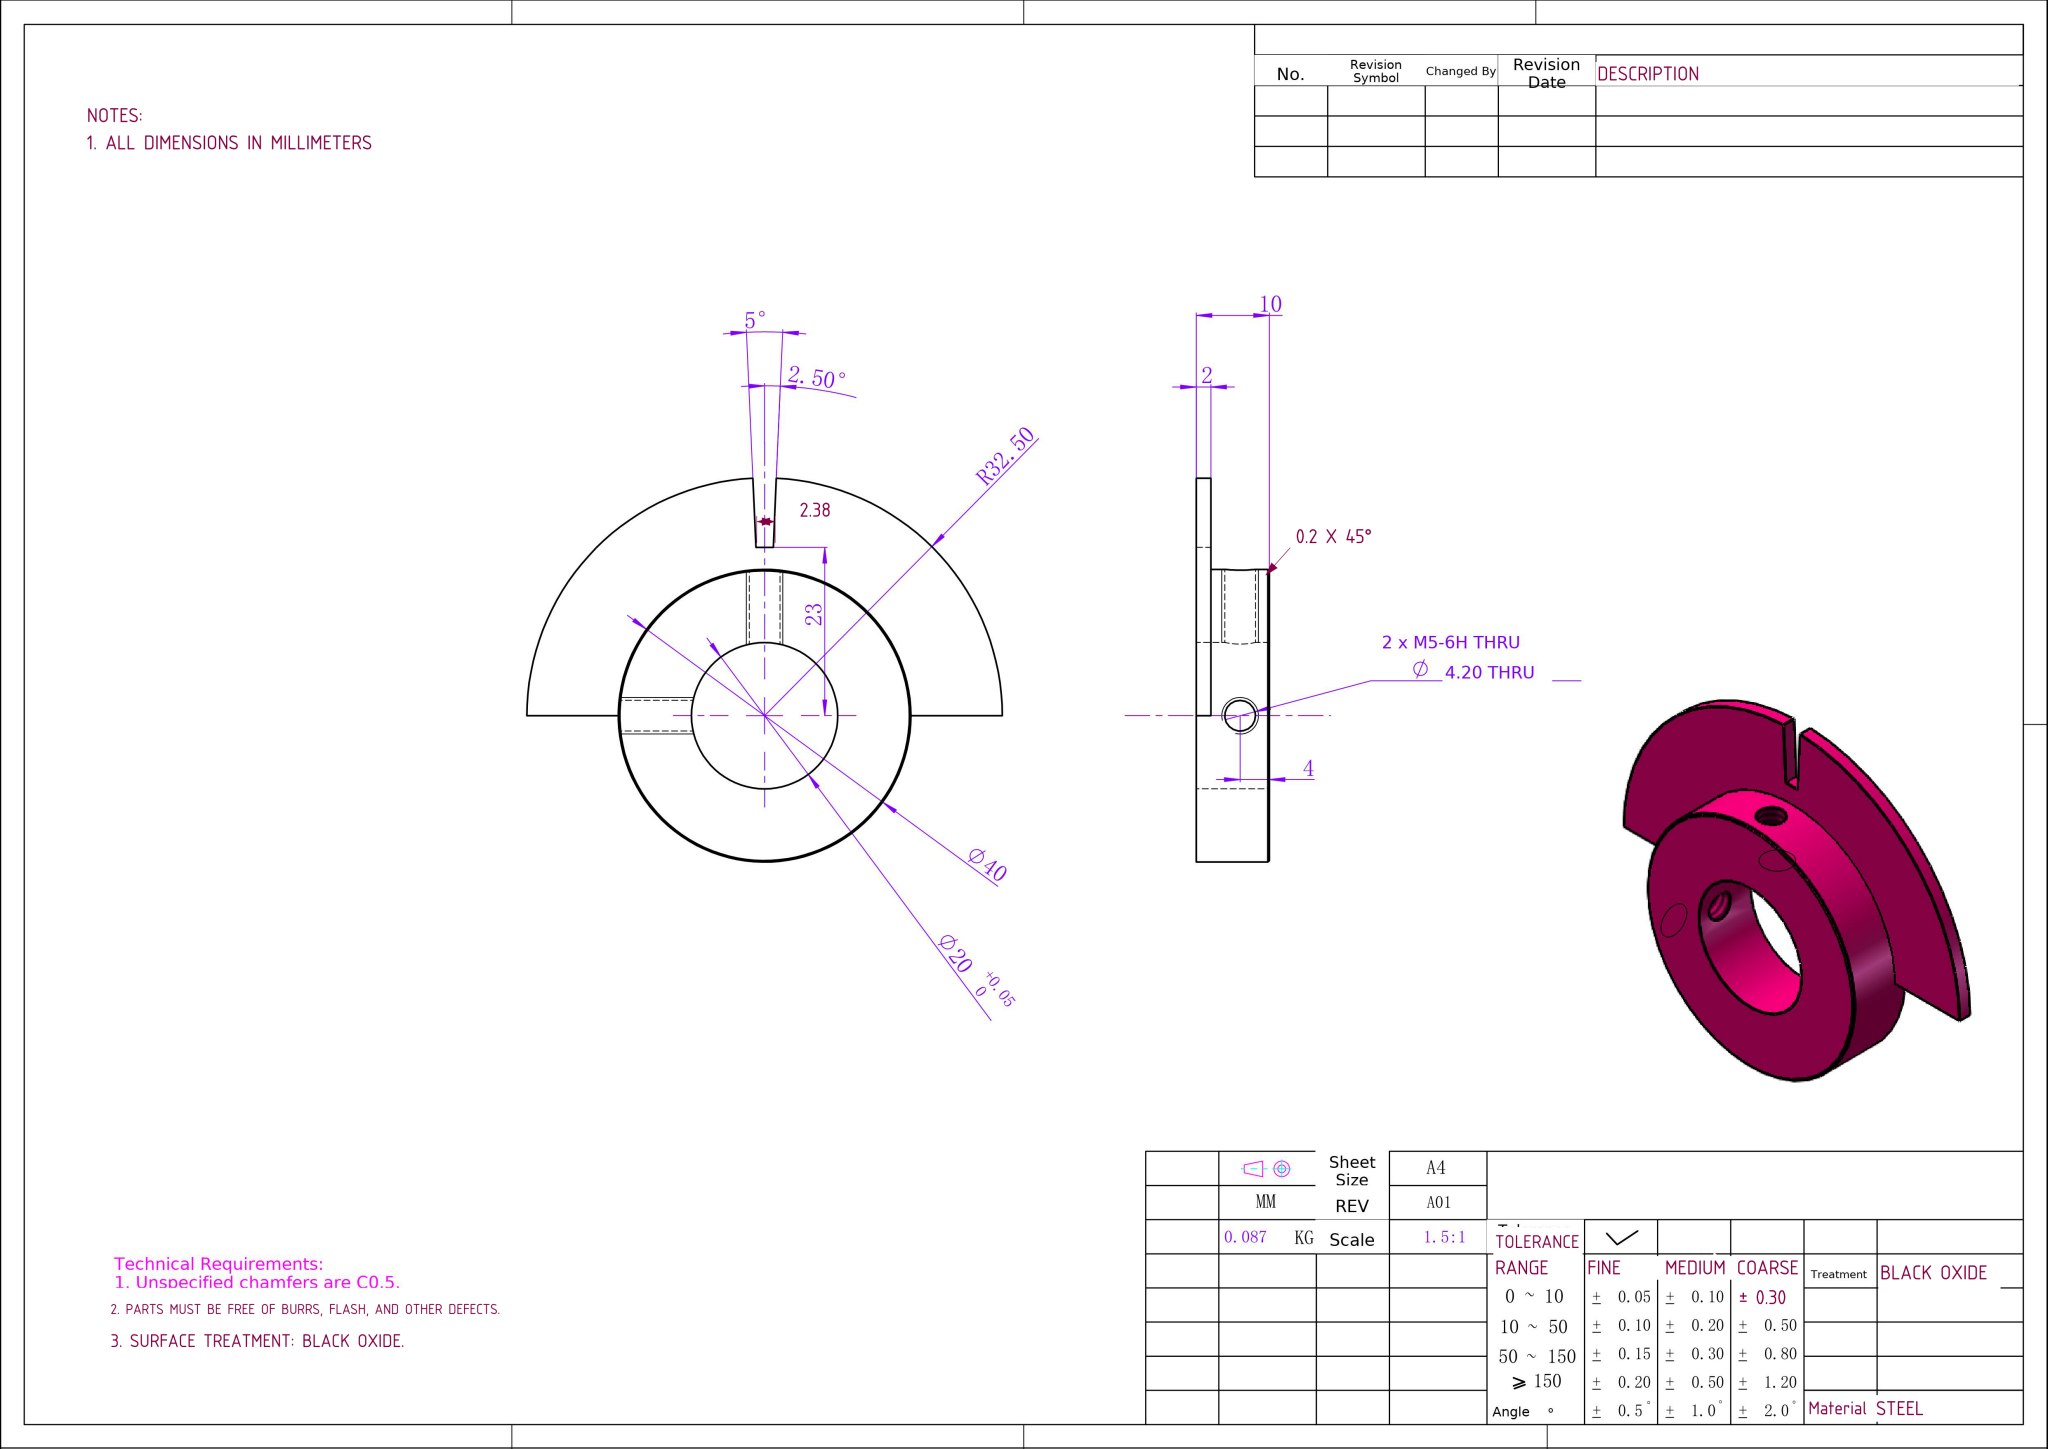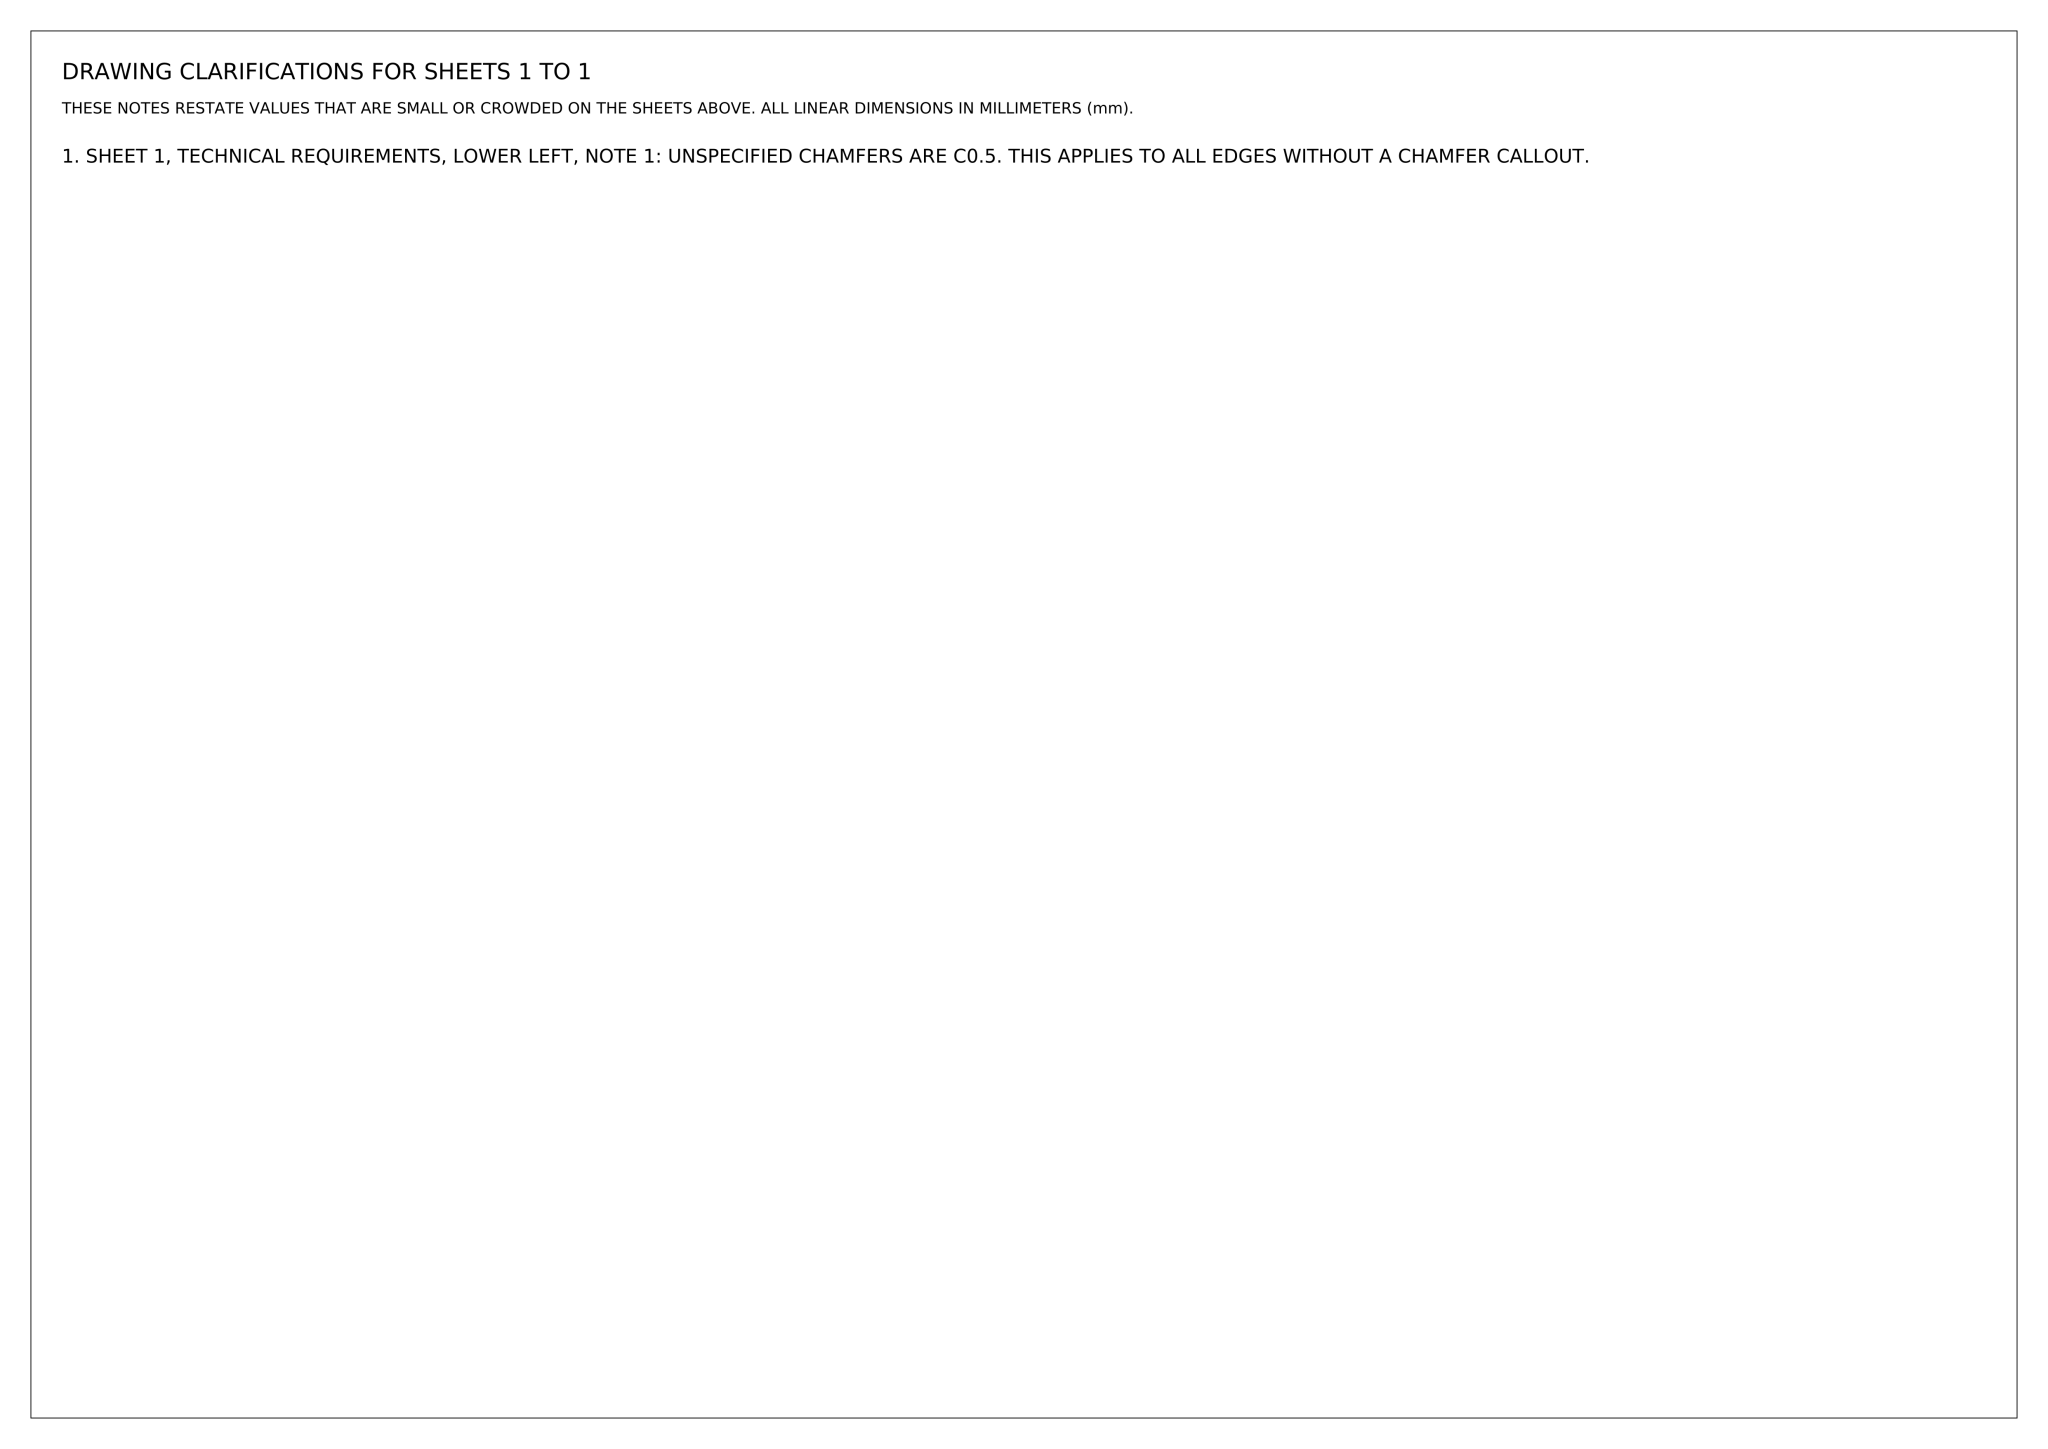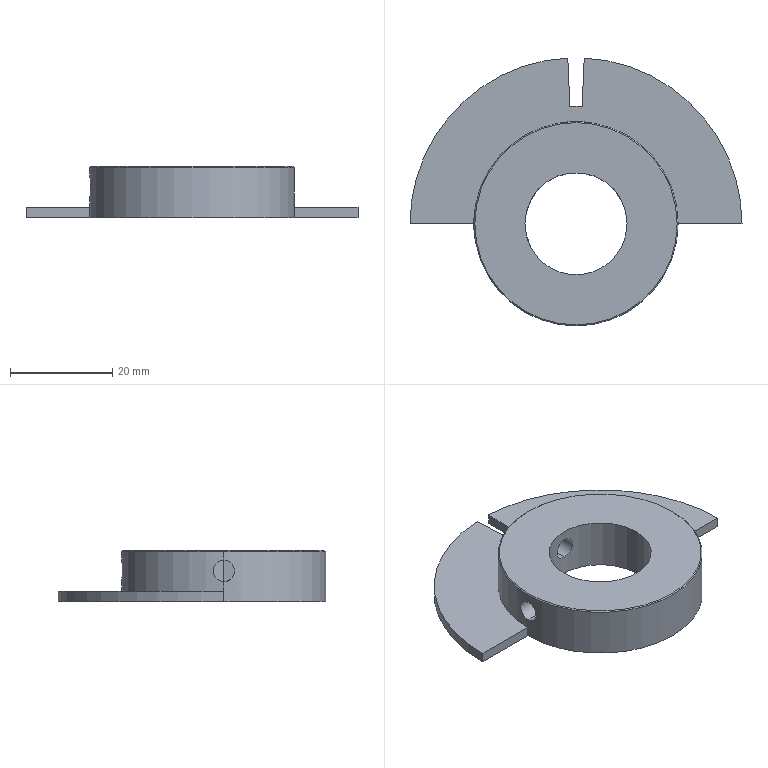Part | NX | mm | 1 solid | 20 faces | box 65 x 52.46 x 10 mm | volume 11153 mm3 | cylinder 10 | plane 8 | cone 2 | commonest cylinder face diameters 4.2 x4 20 x2 40 x2 65 x2